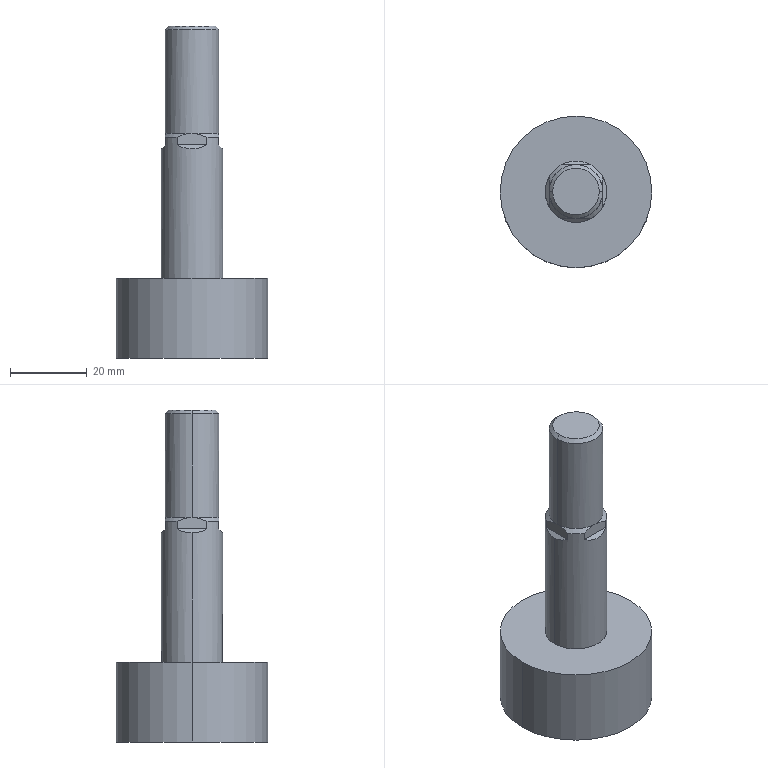Component | SolidWorks | SDA40x20SB_0_+_-1-1_SDAS-40x20-B20_r-1-dx-1 | 1 solid | 23 faces | volume 37279 mm3 | plane 11 | cylinder 6 | cone 6 | commonest cylinder face diameters 39.5 x2 16 x2 14 x2